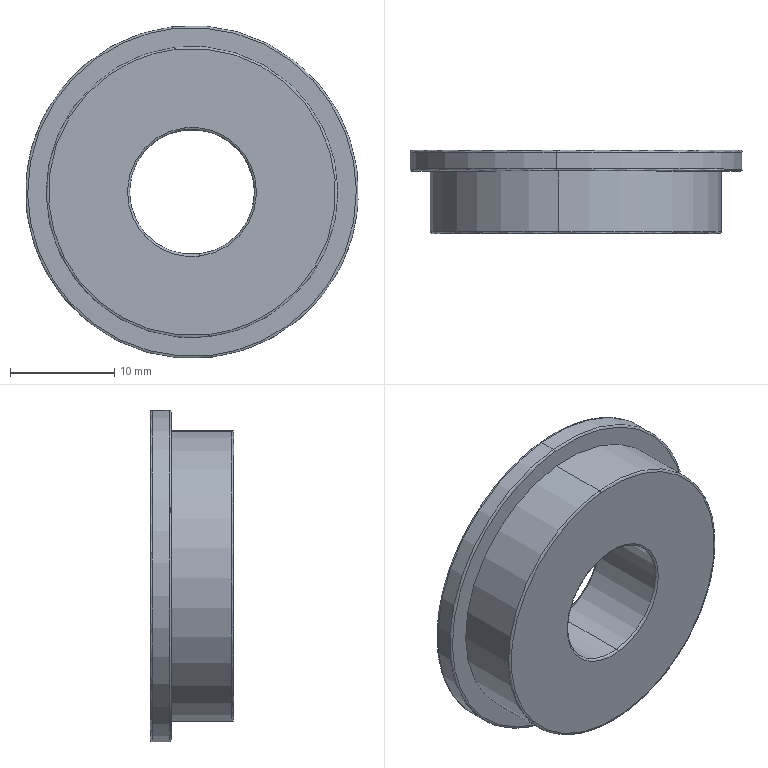Component | SolidWorks | F6001ZZ-11 | 1 solid | 19 faces | volume 4395 mm3 | spline 10 | cylinder 6 | plane 3 | commonest cylinder face diameters 12 x2 32 x2 28 x2